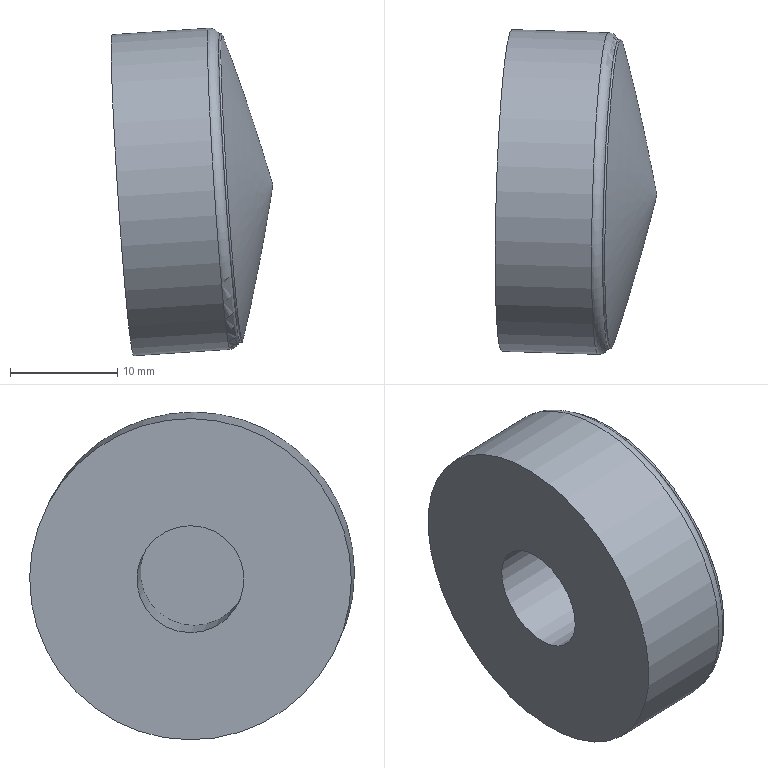Component | NX | CAP2_2 | 2 solids | 8 faces | box 15.34 x 30.27 x 30.53 mm | volume 7279 mm3 | plane 3 | cylinder 2 | torus 2 | other 1 | commonest cylinder face diameters 30 x1 10 x1
STEP:
#1=CARTESIAN_POINT('',(0.,0.,0.));
#2=DIRECTION('',(0.,0.,1.));
#3=DIRECTION('',(1.,0.,0.));
#4=AXIS2_PLACEMENT_3D('',#1,#2,#3);
#5=CARTESIAN_POINT('',(302.238,-314.27,270.967));
#6=VERTEX_POINT('',#5);
#7=CARTESIAN_POINT('',(301.14,-321.165,284.243));
#8=DIRECTION('',(-0.9973,0.03139,-0.06617));
#9=DIRECTION('',(0.07319,0.4597,-0.885));
#10=AXIS2_PLACEMENT_3D('',#7,#8,#9);
#11=CIRCLE('',#10,15.);
#12=CARTESIAN_POINT('',(302.138,-321.197,284.309));
#13=DIRECTION('',(-0.9973,0.03139,-0.06617));
#14=DIRECTION('',(-0.07319,-0.4597,0.885));
#15=AXIS2_PLACEMENT_3D('',#12,#13,#14);
#16=CYLINDRICAL_SURFACE('',#15,15.);
#17=CARTESIAN_POINT('',(3.142,1.));
#18=DIRECTION('',(1.,0.));
#19=VECTOR('',#18,1.);
#20=LINE('',#17,#19);
#21=(GEOMETRIC_REPRESENTATION_CONTEXT(2)PARAMETRIC_REPRESENTATION_CONTEXT()REPRESENTATION_CONTEXT('',''));
#22=DEFINITIONAL_REPRESENTATION('',(#20),#21);
#23=PCURVE('',#16,#22);
#24=CARTESIAN_POINT('',(301.14,-321.165,284.243));
#25=DIRECTION('',(0.9973,-0.03139,0.06617));
#26=DIRECTION('',(0.07319,0.4597,-0.885));
#27=AXIS2_PLACEMENT_3D('',#24,#25,#26);
#28=TOROIDAL_SURFACE('',#27,14.,1.);
#29=CARTESIAN_POINT('',(6.283,6.283));
#30=DIRECTION('',(-1.,0.));
#31=VECTOR('',#30,1.);
#32=LINE('',#29,#31);
#33=(GEOMETRIC_REPRESENTATION_CONTEXT(2)PARAMETRIC_REPRESENTATION_CONTEXT()REPRESENTATION_CONTEXT('',''));
#34=DEFINITIONAL_REPRESENTATION('',(#32),#33);
#35=PCURVE('',#28,#34);
#36=SURFACE_CURVE('',#11,(#23,#35),.PCURVE_S1.);
#37=EDGE_CURVE('',#6,#6,#36,.T.);
#38=ORIENTED_EDGE('',*,*,#37,.T.);
#39=CARTESIAN_POINT('',(293.262,-313.987,270.372));
#40=VERTEX_POINT('',#39);
#41=CARTESIAN_POINT('',(302.238,-314.27,270.967));
#42=CARTESIAN_POINT('',(293.262,-313.987,270.372));
#43=B_SPLINE_CURVE_WITH_KNOTS('',1,(#41,#42),.UNSPECIFIED.,.F.,.F.,(2,2),(1.,10.),.PIECEWISE_BEZIER_KNOTS.);
#44=CARTESIAN_POINT('',(9.425,0.));
#45=DIRECTION('',(0.,1.));
#46=VECTOR('',#45,1.);
#47=LINE('',#44,#46);
#48=(GEOMETRIC_REPRESENTATION_CONTEXT(2)PARAMETRIC_REPRESENTATION_CONTEXT()REPRESENTATION_CONTEXT('',''));
#49=DEFINITIONAL_REPRESENTATION('',(#47),#48);
#50=PCURVE('',#16,#49);
#51=CARTESIAN_POINT('',(3.142,0.));
#52=DIRECTION('',(0.,1.));
#53=VECTOR('',#52,1.);
#54=LINE('',#51,#53);
#55=(GEOMETRIC_REPRESENTATION_CONTEXT(2)PARAMETRIC_REPRESENTATION_CONTEXT()REPRESENTATION_CONTEXT('',''));
#56=DEFINITIONAL_REPRESENTATION('',(#54),#55);
#57=PCURVE('',#16,#56);
#58=SEAM_CURVE('',#43,(#50,#57),.PCURVE_S1.);
#59=EDGE_CURVE('',#6,#40,#58,.T.);
#60=ORIENTED_EDGE('',*,*,#59,.T.);
#61=CARTESIAN_POINT('',(292.165,-320.883,283.648));
#62=DIRECTION('',(0.9973,-0.03139,0.06617));
#63=DIRECTION('',(0.07319,0.4597,-0.885));
#64=AXIS2_PLACEMENT_3D('',#61,#62,#63);
#65=CIRCLE('',#64,15.);
#66=CARTESIAN_POINT('',(9.425,10.));
#67=DIRECTION('',(-1.,0.));
#68=VECTOR('',#67,1.);
#69=LINE('',#66,#68);
#70=(GEOMETRIC_REPRESENTATION_CONTEXT(2)PARAMETRIC_REPRESENTATION_CONTEXT()REPRESENTATION_CONTEXT('',''));
#71=DEFINITIONAL_REPRESENTATION('',(#69),#70);
#72=PCURVE('',#16,#71);
#73=CARTESIAN_POINT('',(292.165,-320.883,283.648));
#74=DIRECTION('',(0.9973,-0.03139,0.06617));
#75=DIRECTION('',(0.07319,0.4597,-0.885));
#76=AXIS2_PLACEMENT_3D('',#73,#74,#75);
#77=PLANE('',#76);
#78=CARTESIAN_POINT('',(0.,0.));
#79=DIRECTION('',(1.,0.));
#80=AXIS2_PLACEMENT_2D('',#78,#79);
#81=CIRCLE('',#80,15.);
#82=(GEOMETRIC_REPRESENTATION_CONTEXT(2)PARAMETRIC_REPRESENTATION_CONTEXT()REPRESENTATION_CONTEXT('',''));
#83=DEFINITIONAL_REPRESENTATION('',(#81),#82);
#84=PCURVE('',#77,#83);
#85=SURFACE_CURVE('',#65,(#72,#84),.PCURVE_S1.);
#86=EDGE_CURVE('',#40,#40,#85,.T.);
#87=ORIENTED_EDGE('',*,*,#86,.T.);
#88=ORIENTED_EDGE('',*,*,#59,.F.);
#89=EDGE_LOOP('',(#38,#60,#87,#88));
#90=FACE_BOUND('',#89,.T.);
#91=ADVANCED_FACE('',(#90),#16,.T.);
#92=CARTESIAN_POINT('',(302.504,-318.898,279.884));
#93=VERTEX_POINT('',#92);
#94=CARTESIAN_POINT('',(302.138,-321.197,284.309));
#95=DIRECTION('',(0.9973,-0.03139,0.06617));
#96=DIRECTION('',(0.07319,0.4597,-0.885));
#97=AXIS2_PLACEMENT_3D('',#94,#95,#96);
#98=CIRCLE('',#97,5.);
#99=CARTESIAN_POINT('',(302.138,-321.197,284.309));
#100=DIRECTION('',(0.9973,-0.03139,0.06617));
#101=DIRECTION('',(0.07319,0.4597,-0.885));
#102=AXIS2_PLACEMENT_3D('',#99,#100,#101);
#103=PLANE('',#102);
#104=CARTESIAN_POINT('',(0.,0.));
#105=DIRECTION('',(1.,0.));
#106=AXIS2_PLACEMENT_2D('',#104,#105);
#107=CIRCLE('',#106,5.);
#108=(GEOMETRIC_REPRESENTATION_CONTEXT(2)PARAMETRIC_REPRESENTATION_CONTEXT()REPRESENTATION_CONTEXT('',''));
#109=DEFINITIONAL_REPRESENTATION('',(#107),#108);
#110=PCURVE('',#103,#109);
#111=CARTESIAN_POINT('',(291.167,-320.851,283.581));
#112=DIRECTION('',(0.9973,-0.03139,0.06617));
#113=DIRECTION('',(0.07319,0.4597,-0.885));
#114=AXIS2_PLACEMENT_3D('',#111,#112,#113);
#115=CYLINDRICAL_SURFACE('',#114,5.);
#116=CARTESIAN_POINT('',(0.,11.));
#117=DIRECTION('',(1.,0.));
#118=VECTOR('',#117,1.);
#119=LINE('',#116,#118);
#120=(GEOMETRIC_REPRESENTATION_CONTEXT(2)PARAMETRIC_REPRESENTATION_CONTEXT()REPRESENTATION_CONTEXT('',''));
#121=DEFINITIONAL_REPRESENTATION('',(#119),#120);
#122=PCURVE('',#115,#121);
#123=SURFACE_CURVE('',#98,(#110,#122),.PCURVE_S1.);
#124=EDGE_CURVE('',#93,#93,#123,.T.);
#125=ORIENTED_EDGE('',*,*,#124,.F.);
#126=EDGE_LOOP('',(#125));
#127=FACE_BOUND('',#126,.T.);
#128=CARTESIAN_POINT('',(303.162,-314.761,271.919));
#129=VERTEX_POINT('',#128);
#130=CARTESIAN_POINT('',(302.138,-321.197,284.309));
#131=DIRECTION('',(0.9973,-0.03139,0.06617));
#132=DIRECTION('',(0.07319,0.4597,-0.885));
#133=AXIS2_PLACEMENT_3D('',#130,#131,#132);
#134=CIRCLE('',#133,14.);
#135=CARTESIAN_POINT('',(0.,0.));
#136=DIRECTION('',(1.,0.));
#137=AXIS2_PLACEMENT_2D('',#135,#136);
#138=CIRCLE('',#137,14.);
#139=(GEOMETRIC_REPRESENTATION_CONTEXT(2)PARAMETRIC_REPRESENTATION_CONTEXT()REPRESENTATION_CONTEXT('',''));
#140=DEFINITIONAL_REPRESENTATION('',(#138),#139);
#141=PCURVE('',#103,#140);
#142=CARTESIAN_POINT('',(0.,7.854));
#143=DIRECTION('',(1.,0.));
#144=VECTOR('',#143,1.);
#145=LINE('',#142,#144);
#146=(GEOMETRIC_REPRESENTATION_CONTEXT(2)PARAMETRIC_REPRESENTATION_CONTEXT()REPRESENTATION_CONTEXT('',''));
#147=DEFINITIONAL_REPRESENTATION('',(#145),#146);
#148=PCURVE('',#28,#147);
#149=SURFACE_CURVE('',#134,(#141,#148),.PCURVE_S1.);
#150=EDGE_CURVE('',#129,#129,#149,.T.);
#151=ORIENTED_EDGE('',*,*,#150,.T.);
#152=EDGE_LOOP('',(#151));
#153=FACE_BOUND('',#152,.T.);
#154=ADVANCED_FACE('',(#127,#153),#103,.T.);
#155=CARTESIAN_POINT('',(291.799,-323.181,288.073));
#156=VERTEX_POINT('',#155);
#157=CARTESIAN_POINT('',(292.53,-318.584,279.222));
#158=VERTEX_POINT('',#157);
#159=CARTESIAN_POINT('',(292.165,-320.883,283.648));
#160=DIRECTION('',(-0.9973,0.03139,-0.06617));
#161=DIRECTION('',(-0.07319,-0.4597,0.885));
#162=AXIS2_PLACEMENT_3D('',#159,#160,#161);
#163=CIRCLE('',#162,5.);
#164=CARTESIAN_POINT('',(-5.,-0.));
#165=CARTESIAN_POINT('',(-5.,8.66));
#166=CARTESIAN_POINT('',(2.5,4.33));
#167=CARTESIAN_POINT('',(10.,0.));
#168=CARTESIAN_POINT('',(2.5,-4.33));
#169=CARTESIAN_POINT('',(-5.,-8.66));
#170=CARTESIAN_POINT('',(-5.,-0.));
#171=(BOUNDED_CURVE()B_SPLINE_CURVE(2,(#164,#165,#166,#167,#168,#169,#170),.UNSPECIFIED.,.T.,.F.)B_SPLINE_CURVE_WITH_KNOTS((1,2,2,2,2,1),(-2.094,0.,2.094,4.189,6.283,8.378),.UNSPECIFIED.)CURVE()GEOMETRIC_REPRESENTATION_ITEM()RATIONAL_B_SPLINE_CURVE((1.,0.5,1.,0.5,1.,0.5,1.))REPRESENTATION_ITEM(''));
#172=(GEOMETRIC_REPRESENTATION_CONTEXT(2)PARAMETRIC_REPRESENTATION_CONTEXT()REPRESENTATION_CONTEXT('',''));
#173=DEFINITIONAL_REPRESENTATION('',(#171),#172);
#174=PCURVE('',#77,#173);
#175=CARTESIAN_POINT('',(3.142,1.));
#176=DIRECTION('',(-1.,0.));
#177=VECTOR('',#176,1.);
#178=LINE('',#175,#177);
#179=(GEOMETRIC_REPRESENTATION_CONTEXT(2)PARAMETRIC_REPRESENTATION_CONTEXT()REPRESENTATION_CONTEXT('',''));
#180=DEFINITIONAL_REPRESENTATION('',(#178),#179);
#181=PCURVE('',#115,#180);
#182=SURFACE_CURVE('',#163,(#174,#181),.PCURVE_S1.);
#183=EDGE_CURVE('',#156,#158,#182,.T.);
#184=ORIENTED_EDGE('',*,*,#183,.F.);
#185=CARTESIAN_POINT('',(292.165,-320.883,283.648));
#186=DIRECTION('',(-0.9973,0.03139,-0.06617));
#187=DIRECTION('',(-0.07319,-0.4597,0.885));
#188=AXIS2_PLACEMENT_3D('',#185,#186,#187);
#189=CIRCLE('',#188,5.);
#190=CARTESIAN_POINT('',(-5.,-0.));
#191=CARTESIAN_POINT('',(-5.,8.66));
#192=CARTESIAN_POINT('',(2.5,4.33));
#193=CARTESIAN_POINT('',(10.,0.));
#194=CARTESIAN_POINT('',(2.5,-4.33));
#195=CARTESIAN_POINT('',(-5.,-8.66));
#196=CARTESIAN_POINT('',(-5.,-0.));
#197=(BOUNDED_CURVE()B_SPLINE_CURVE(2,(#190,#191,#192,#193,#194,#195,#196),.UNSPECIFIED.,.T.,.F.)B_SPLINE_CURVE_WITH_KNOTS((1,2,2,2,2,1),(-2.094,0.,2.094,4.189,6.283,8.378),.UNSPECIFIED.)CURVE()GEOMETRIC_REPRESENTATION_ITEM()RATIONAL_B_SPLINE_CURVE((1.,0.5,1.,0.5,1.,0.5,1.))REPRESENTATION_ITEM(''));
#198=(GEOMETRIC_REPRESENTATION_CONTEXT(2)PARAMETRIC_REPRESENTATION_CONTEXT()REPRESENTATION_CONTEXT('',''));
#199=DEFINITIONAL_REPRESENTATION('',(#197),#198);
#200=PCURVE('',#77,#199);
#201=CARTESIAN_POINT('',(9.425,1.));
#202=DIRECTION('',(-1.,0.));
#203=VECTOR('',#202,1.);
#204=LINE('',#201,#203);
#205=(GEOMETRIC_REPRESENTATION_CONTEXT(2)PARAMETRIC_REPRESENTATION_CONTEXT()REPRESENTATION_CONTEXT('',''));
#206=DEFINITIONAL_REPRESENTATION('',(#204),#205);
#207=PCURVE('',#115,#206);
#208=SURFACE_CURVE('',#189,(#200,#207),.PCURVE_S1.);
#209=EDGE_CURVE('',#158,#156,#208,.T.);
#210=ORIENTED_EDGE('',*,*,#209,.F.);
#211=EDGE_LOOP('',(#184,#210));
#212=FACE_BOUND('',#211,.T.);
#213=ORIENTED_EDGE('',*,*,#86,.F.);
#214=EDGE_LOOP('',(#213));
#215=FACE_BOUND('',#214,.T.);
#216=ADVANCED_FACE('',(#212,#215),#77,.F.);
#217=ORIENTED_EDGE('',*,*,#37,.F.);
#218=CARTESIAN_POINT('',(302.238,-314.27,270.967));
#219=CARTESIAN_POINT('',(302.505,-314.278,270.985));
#220=CARTESIAN_POINT('',(302.758,-314.325,271.078));
#221=CARTESIAN_POINT('',(302.97,-314.407,271.237));
#222=CARTESIAN_POINT('',(303.116,-314.515,271.446));
#223=CARTESIAN_POINT('',(303.182,-314.638,271.682));
#224=CARTESIAN_POINT('',(303.162,-314.761,271.919));
#225=(BOUNDED_CURVE()B_SPLINE_CURVE(6,(#218,#219,#220,#221,#222,#223,#224),.UNSPECIFIED.,.F.,.F.)B_SPLINE_CURVE_WITH_KNOTS((7,7),(0.,1.571),.PIECEWISE_BEZIER_KNOTS.)CURVE()GEOMETRIC_REPRESENTATION_ITEM()RATIONAL_B_SPLINE_CURVE((1.031,1.01,0.9979,0.994,0.9979,1.01,1.031))REPRESENTATION_ITEM(''));
#226=CARTESIAN_POINT('',(6.283,6.283));
#227=DIRECTION('',(0.,1.));
#228=VECTOR('',#227,1.);
#229=LINE('',#226,#228);
#230=(GEOMETRIC_REPRESENTATION_CONTEXT(2)PARAMETRIC_REPRESENTATION_CONTEXT()REPRESENTATION_CONTEXT('',''));
#231=DEFINITIONAL_REPRESENTATION('',(#229),#230);
#232=PCURVE('',#28,#231);
#233=CARTESIAN_POINT('',(0.,6.283));
#234=DIRECTION('',(0.,1.));
#235=VECTOR('',#234,1.);
#236=LINE('',#233,#235);
#237=(GEOMETRIC_REPRESENTATION_CONTEXT(2)PARAMETRIC_REPRESENTATION_CONTEXT()REPRESENTATION_CONTEXT('',''));
#238=DEFINITIONAL_REPRESENTATION('',(#236),#237);
#239=PCURVE('',#28,#238);
#240=SEAM_CURVE('',#225,(#232,#239),.PCURVE_S1.);
#241=EDGE_CURVE('',#6,#129,#240,.T.);
#242=ORIENTED_EDGE('',*,*,#241,.T.);
#243=ORIENTED_EDGE('',*,*,#150,.F.);
#244=ORIENTED_EDGE('',*,*,#241,.F.);
#245=EDGE_LOOP('',(#217,#242,#243,#244));
#246=FACE_BOUND('',#245,.T.);
#247=ADVANCED_FACE('',(#246),#28,.T.);
#248=ORIENTED_EDGE('',*,*,#209,.F.);
#249=CARTESIAN_POINT('',(292.53,-318.584,279.222));
#250=CARTESIAN_POINT('',(302.504,-318.898,279.884));
#251=B_SPLINE_CURVE_WITH_KNOTS('',1,(#249,#250),.UNSPECIFIED.,.F.,.F.,(2,2),(1.,11.),.PIECEWISE_BEZIER_KNOTS.);
#252=CARTESIAN_POINT('',(6.283,0.));
#253=DIRECTION('',(0.,1.));
#254=VECTOR('',#253,1.);
#255=LINE('',#252,#254);
#256=(GEOMETRIC_REPRESENTATION_CONTEXT(2)PARAMETRIC_REPRESENTATION_CONTEXT()REPRESENTATION_CONTEXT('',''));
#257=DEFINITIONAL_REPRESENTATION('',(#255),#256);
#258=PCURVE('',#115,#257);
#259=CARTESIAN_POINT('',(0.,0.));
#260=DIRECTION('',(0.,1.));
#261=VECTOR('',#260,1.);
#262=LINE('',#259,#261);
#263=(GEOMETRIC_REPRESENTATION_CONTEXT(2)PARAMETRIC_REPRESENTATION_CONTEXT()REPRESENTATION_CONTEXT('',''));
#264=DEFINITIONAL_REPRESENTATION('',(#262),#263);
#265=PCURVE('',#115,#264);
#266=SEAM_CURVE('',#251,(#258,#265),.PCURVE_S1.);
#267=EDGE_CURVE('',#158,#93,#266,.T.);
#268=ORIENTED_EDGE('',*,*,#267,.T.);
#269=ORIENTED_EDGE('',*,*,#124,.F.);
#270=ORIENTED_EDGE('',*,*,#267,.F.);
#271=ORIENTED_EDGE('',*,*,#183,.F.);
#272=EDGE_LOOP('',(#248,#268,#269,#270,#271));
#273=FACE_BOUND('',#272,.F.);
#274=ADVANCED_FACE('',(#273),#115,.F.);
#275=CLOSED_SHELL('',(#91,#154,#216,#247,#274));
#276=MANIFOLD_SOLID_BREP('',#275);
#277=(LENGTH_UNIT()NAMED_UNIT(*)SI_UNIT(.MILLI.,.METRE.));
#278=UNCERTAINTY_MEASURE_WITH_UNIT(LENGTH_MEASURE(0.000005),#277,'','');
#279=(NAMED_UNIT(*)PLANE_ANGLE_UNIT()SI_UNIT($,.RADIAN.));
#280=(NAMED_UNIT(*)SI_UNIT($,.STERADIAN.)SOLID_ANGLE_UNIT());
#281=(GEOMETRIC_REPRESENTATION_CONTEXT(3)GLOBAL_UNCERTAINTY_ASSIGNED_CONTEXT((#278))GLOBAL_UNIT_ASSIGNED_CONTEXT((#277,#279,#280))REPRESENTATION_CONTEXT('',''));
#282=ADVANCED_BREP_SHAPE_REPRESENTATION('',(#4,#276),#281);
#283=CARTESIAN_POINT('',(0.,0.,0.));
#284=DIRECTION('',(0.,0.,1.));
#285=DIRECTION('',(1.,0.,0.));
#286=AXIS2_PLACEMENT_3D('',#283,#284,#285);
#287=CARTESIAN_POINT('',(0.,0.,0.));
#288=DIRECTION('',(0.,0.,1.));
#289=DIRECTION('',(1.,0.,0.));
#290=AXIS2_PLACEMENT_3D('',#287,#288,#289);
#291=(LENGTH_UNIT()NAMED_UNIT(*)SI_UNIT(.MILLI.,.METRE.));
#292=UNCERTAINTY_MEASURE_WITH_UNIT(LENGTH_MEASURE(0.00001),#291,'','');
#293=(NAMED_UNIT(*)PLANE_ANGLE_UNIT()SI_UNIT($,.RADIAN.));
#294=(NAMED_UNIT(*)SI_UNIT($,.STERADIAN.)SOLID_ANGLE_UNIT());
#295=(GEOMETRIC_REPRESENTATION_CONTEXT(3)GLOBAL_UNCERTAINTY_ASSIGNED_CONTEXT((#292))GLOBAL_UNIT_ASSIGNED_CONTEXT((#291,#293,#294))REPRESENTATION_CONTEXT('',''));
#296=SHAPE_REPRESENTATION('',(#4,#286,#290),#295);
#297=ITEM_DEFINED_TRANSFORMATION('','',#4,#286);
#298=(REPRESENTATION_RELATIONSHIP('','',#282,#296)REPRESENTATION_RELATIONSHIP_WITH_TRANSFORMATION(#297)SHAPE_REPRESENTATION_RELATIONSHIP());
#299=CARTESIAN_POINT('',(303.187,-314.604,271.616));
#300=VERTEX_POINT('',#299);
#301=CARTESIAN_POINT('',(302.138,-321.197,284.309));
#302=DIRECTION('',(-0.9973,0.03139,-0.06617));
#303=DIRECTION('',(0.07319,0.4597,-0.885));
#304=AXIS2_PLACEMENT_3D('',#301,#302,#303);
#305=CIRCLE('',#304,14.341);
#306=CARTESIAN_POINT('',(302.138,-321.197,284.309));
#307=DIRECTION('',(0.9973,-0.03139,0.06617));
#308=DIRECTION('',(0.07319,0.4597,-0.885));
#309=AXIS2_PLACEMENT_3D('',#306,#307,#308);
#310=PLANE('',#309);
#311=CARTESIAN_POINT('',(14.341,-0.));
#312=CARTESIAN_POINT('',(14.341,-24.84));
#313=CARTESIAN_POINT('',(-7.171,-12.42));
#314=CARTESIAN_POINT('',(-28.683,-0.));
#315=CARTESIAN_POINT('',(-7.171,12.42));
#316=CARTESIAN_POINT('',(14.341,24.84));
#317=CARTESIAN_POINT('',(14.341,-0.));
#318=(BOUNDED_CURVE()B_SPLINE_CURVE(2,(#311,#312,#313,#314,#315,#316,#317),.UNSPECIFIED.,.T.,.F.)B_SPLINE_CURVE_WITH_KNOTS((1,2,2,2,2,1),(-2.094,0.,2.094,4.189,6.283,8.378),.UNSPECIFIED.)CURVE()GEOMETRIC_REPRESENTATION_ITEM()RATIONAL_B_SPLINE_CURVE((1.,0.5,1.,0.5,1.,0.5,1.))REPRESENTATION_ITEM(''));
#319=(GEOMETRIC_REPRESENTATION_CONTEXT(2)PARAMETRIC_REPRESENTATION_CONTEXT()REPRESENTATION_CONTEXT('',''));
#320=DEFINITIONAL_REPRESENTATION('',(#318),#319);
#321=PCURVE('',#310,#320);
#322=CARTESIAN_POINT('',(302.237,-321.2,284.316));
#323=DIRECTION('',(0.9973,-0.03139,0.06617));
#324=DIRECTION('',(0.07319,0.4597,-0.885));
#325=AXIS2_PLACEMENT_3D('',#322,#323,#324);
#326=TOROIDAL_SURFACE('',#325,14.341,0.1);
#327=CARTESIAN_POINT('',(6.283,4.712));
#328=DIRECTION('',(-1.,0.));
#329=VECTOR('',#328,1.);
#330=LINE('',#327,#329);
#331=(GEOMETRIC_REPRESENTATION_CONTEXT(2)PARAMETRIC_REPRESENTATION_CONTEXT()REPRESENTATION_CONTEXT('',''));
#332=DEFINITIONAL_REPRESENTATION('',(#330),#331);
#333=PCURVE('',#326,#332);
#334=SURFACE_CURVE('',#305,(#321,#333),.PCURVE_S1.);
#335=EDGE_CURVE('',#300,#300,#334,.T.);
#336=ORIENTED_EDGE('',*,*,#335,.T.);
#337=EDGE_LOOP('',(#336));
#338=FACE_BOUND('',#337,.T.);
#339=ADVANCED_FACE('',(#338),#310,.F.);
#340=CARTESIAN_POINT('',(303.384,-314.596,271.603));
#341=VERTEX_POINT('',#340);
#342=CARTESIAN_POINT('',(302.333,-321.203,284.322));
#343=DIRECTION('',(0.9973,-0.03139,0.06617));
#344=DIRECTION('',(0.07319,0.4597,-0.885));
#345=AXIS2_PLACEMENT_3D('',#342,#343,#344);
#346=CIRCLE('',#345,14.371);
#347=CARTESIAN_POINT('',(303.384,-314.596,271.603));
#348=CARTESIAN_POINT('',(304.972,-317.772,277.729));
#349=CARTESIAN_POINT('',(306.127,-321.322,284.574));
#350=(BOUNDED_CURVE()B_SPLINE_CURVE(2,(#347,#348,#349),.UNSPECIFIED.,.F.,.F.)B_SPLINE_CURVE_WITH_KNOTS((3,3),(0.,1.),.PIECEWISE_BEZIER_KNOTS.)CURVE()GEOMETRIC_REPRESENTATION_ITEM()RATIONAL_B_SPLINE_CURVE((0.5,0.5,0.5))REPRESENTATION_ITEM(''));
#351=CARTESIAN_POINT('',(302.138,-321.197,284.309));
#352=DIRECTION('',(0.9973,-0.03139,0.06617));
#353=AXIS1_PLACEMENT('',#351,#352);
#354=SURFACE_OF_REVOLUTION('',#350,#353);
#355=CARTESIAN_POINT('',(0.,0.));
#356=DIRECTION('',(1.,0.));
#357=VECTOR('',#356,1.);
#358=LINE('',#355,#357);
#359=(GEOMETRIC_REPRESENTATION_CONTEXT(2)PARAMETRIC_REPRESENTATION_CONTEXT()REPRESENTATION_CONTEXT('',''));
#360=DEFINITIONAL_REPRESENTATION('',(#358),#359);
#361=PCURVE('',#354,#360);
#362=CARTESIAN_POINT('',(0.,7.555));
#363=DIRECTION('',(1.,0.));
#364=VECTOR('',#363,1.);
#365=LINE('',#362,#364);
#366=(GEOMETRIC_REPRESENTATION_CONTEXT(2)PARAMETRIC_REPRESENTATION_CONTEXT()REPRESENTATION_CONTEXT('',''));
#367=DEFINITIONAL_REPRESENTATION('',(#365),#366);
#368=PCURVE('',#326,#367);
#369=SURFACE_CURVE('',#346,(#361,#368),.PCURVE_S1.);
#370=EDGE_CURVE('',#341,#341,#369,.T.);
#371=ORIENTED_EDGE('',*,*,#370,.T.);
#372=CARTESIAN_POINT('',(306.127,-321.322,284.574));
#373=VERTEX_POINT('',#372);
#374=CARTESIAN_POINT('',(303.384,-314.596,271.603));
#375=CARTESIAN_POINT('',(304.972,-317.772,277.729));
#376=CARTESIAN_POINT('',(306.127,-321.322,284.574));
#377=(BOUNDED_CURVE()B_SPLINE_CURVE(2,(#374,#375,#376),.UNSPECIFIED.,.F.,.F.)B_SPLINE_CURVE_WITH_KNOTS((3,3),(0.,1.),.PIECEWISE_BEZIER_KNOTS.)CURVE()GEOMETRIC_REPRESENTATION_ITEM()RATIONAL_B_SPLINE_CURVE((0.5,0.5,0.5))REPRESENTATION_ITEM(''));
#378=CARTESIAN_POINT('',(6.283,0.));
#379=DIRECTION('',(0.,1.));
#380=VECTOR('',#379,1.);
#381=LINE('',#378,#380);
#382=(GEOMETRIC_REPRESENTATION_CONTEXT(2)PARAMETRIC_REPRESENTATION_CONTEXT()REPRESENTATION_CONTEXT('',''));
#383=DEFINITIONAL_REPRESENTATION('',(#381),#382);
#384=PCURVE('',#354,#383);
#385=CARTESIAN_POINT('',(0.,0.));
#386=DIRECTION('',(0.,1.));
#387=VECTOR('',#386,1.);
#388=LINE('',#385,#387);
#389=(GEOMETRIC_REPRESENTATION_CONTEXT(2)PARAMETRIC_REPRESENTATION_CONTEXT()REPRESENTATION_CONTEXT('',''));
#390=DEFINITIONAL_REPRESENTATION('',(#388),#389);
#391=PCURVE('',#354,#390);
#392=SEAM_CURVE('',#377,(#384,#391),.PCURVE_S1.);
#393=EDGE_CURVE('',#341,#373,#392,.T.);
#394=ORIENTED_EDGE('',*,*,#393,.T.);
#395=ORIENTED_EDGE('',*,*,#393,.F.);
#396=EDGE_LOOP('',(#371,#394,#395));
#397=FACE_BOUND('',#396,.T.);
#398=ADVANCED_FACE('',(#397),#354,.T.);
#399=ORIENTED_EDGE('',*,*,#335,.F.);
#400=CARTESIAN_POINT('',(303.187,-314.604,271.616));
#401=CARTESIAN_POINT('',(303.19,-314.585,271.581));
#402=CARTESIAN_POINT('',(303.212,-314.567,271.546));
#403=CARTESIAN_POINT('',(303.253,-314.555,271.522));
#404=CARTESIAN_POINT('',(303.303,-314.553,271.519));
#405=CARTESIAN_POINT('',(303.348,-314.562,271.537));
#406=CARTESIAN_POINT('',(303.375,-314.578,271.568));
#407=CARTESIAN_POINT('',(303.384,-314.596,271.603));
#408=B_SPLINE_CURVE_WITH_KNOTS('',7,(#400,#401,#402,#403,#404,#405,#406,#407),.UNSPECIFIED.,.F.,.F.,(8,8),(4.712,7.555),.PIECEWISE_BEZIER_KNOTS.);
#409=CARTESIAN_POINT('',(6.283,0.));
#410=DIRECTION('',(0.,1.));
#411=VECTOR('',#410,1.);
#412=LINE('',#409,#411);
#413=(GEOMETRIC_REPRESENTATION_CONTEXT(2)PARAMETRIC_REPRESENTATION_CONTEXT()REPRESENTATION_CONTEXT('',''));
#414=DEFINITIONAL_REPRESENTATION('',(#412),#413);
#415=PCURVE('',#326,#414);
#416=CARTESIAN_POINT('',(0.,0.));
#417=DIRECTION('',(0.,1.));
#418=VECTOR('',#417,1.);
#419=LINE('',#416,#418);
#420=(GEOMETRIC_REPRESENTATION_CONTEXT(2)PARAMETRIC_REPRESENTATION_CONTEXT()REPRESENTATION_CONTEXT('',''));
#421=DEFINITIONAL_REPRESENTATION('',(#419),#420);
#422=PCURVE('',#326,#421);
#423=SEAM_CURVE('',#408,(#415,#422),.PCURVE_S1.);
#424=EDGE_CURVE('',#300,#341,#423,.T.);
#425=ORIENTED_EDGE('',*,*,#424,.T.);
#426=ORIENTED_EDGE('',*,*,#370,.F.);
#427=ORIENTED_EDGE('',*,*,#424,.F.);
#428=EDGE_LOOP('',(#399,#425,#426,#427));
#429=FACE_BOUND('',#428,.T.);
#430=ADVANCED_FACE('',(#429),#326,.T.);
#431=CLOSED_SHELL('',(#339,#398,#430));
#432=MANIFOLD_SOLID_BREP('',#431);
#433=(LENGTH_UNIT()NAMED_UNIT(*)SI_UNIT(.MILLI.,.METRE.));
#434=UNCERTAINTY_MEASURE_WITH_UNIT(LENGTH_MEASURE(0.00001),#433,'','');
#435=(NAMED_UNIT(*)PLANE_ANGLE_UNIT()SI_UNIT($,.RADIAN.));
#436=(NAMED_UNIT(*)SI_UNIT($,.STERADIAN.)SOLID_ANGLE_UNIT());
#437=(GEOMETRIC_REPRESENTATION_CONTEXT(3)GLOBAL_UNCERTAINTY_ASSIGNED_CONTEXT((#434))GLOBAL_UNIT_ASSIGNED_CONTEXT((#433,#435,#436))REPRESENTATION_CONTEXT('',''));
#438=ADVANCED_BREP_SHAPE_REPRESENTATION('',(#4,#432),#437);
#439=ITEM_DEFINED_TRANSFORMATION('','',#4,#290);
#440=(REPRESENTATION_RELATIONSHIP('','',#438,#296)REPRESENTATION_RELATIONSHIP_WITH_TRANSFORMATION(#439)SHAPE_REPRESENTATION_RELATIONSHIP());